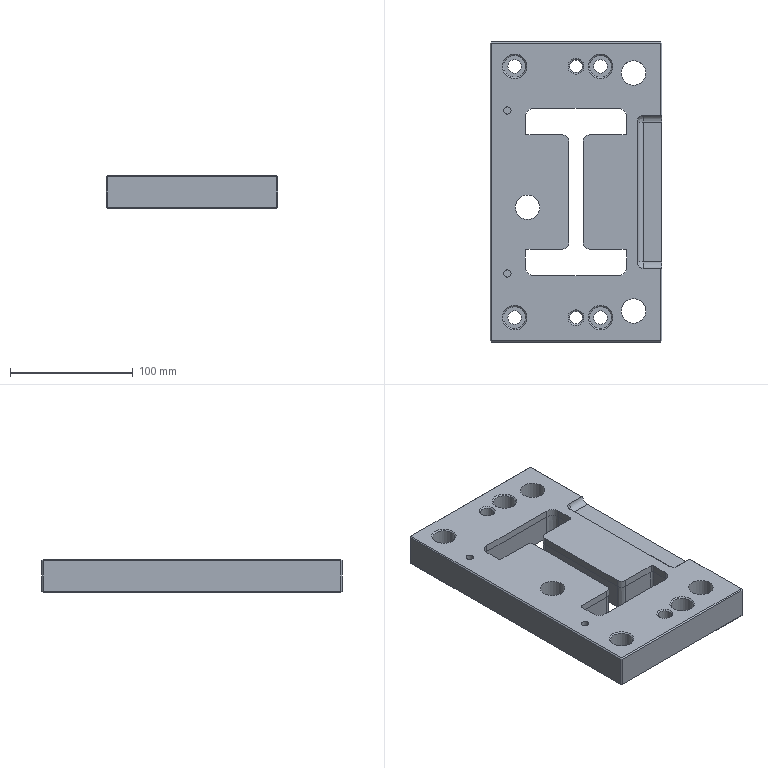Component | NX | DIE | 1 solid | 123 faces | volume 728663 mm3 | plane 63 | cylinder 34 | cone 24 | spline 2 | commonest cylinder face diameters 11 x6 18 x4 6 x4 2.914 x4 10.086 x4 13.914 x4 20.02 x3 10.2 x2